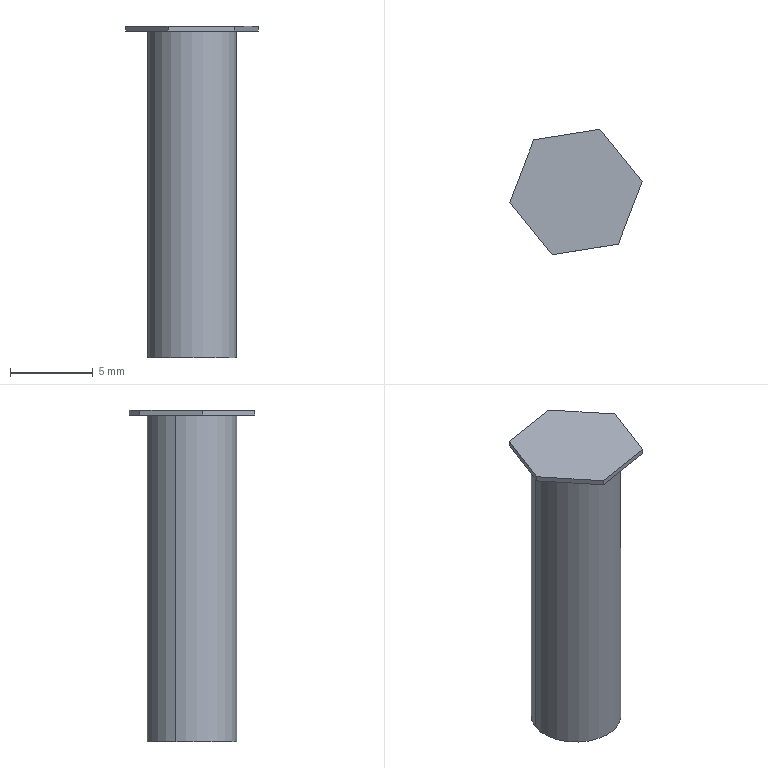Component | SolidWorks | P16BoxWeldment-1_BSO-M3-20-13 | 1 solid | 14 faces | box 7.99 x 7.56 x 20 mm | volume 358 mm3 | plane 10 | cylinder 4 | commonest cylinder face diameters 3 x2 5.4 x2
STEP:
#1=COLOUR_RGB('',0.7922,0.8196,0.9333);
#2=FILL_AREA_STYLE_COLOUR('',#1);
#3=FILL_AREA_STYLE('',(#2));
#4=SURFACE_STYLE_FILL_AREA(#3);
#5=SURFACE_SIDE_STYLE('',(#4));
#6=SURFACE_STYLE_USAGE(.BOTH.,#5);
#7=PRESENTATION_STYLE_ASSIGNMENT((#6));
#8=CARTESIAN_POINT('',(-18.287,3.589,2.535));
#9=VERTEX_POINT('',#8);
#10=CARTESIAN_POINT('',(-18.397,3.632,2.535));
#11=VERTEX_POINT('',#10);
#12=CARTESIAN_POINT('',(-18.342,3.611,2.535));
#13=DIRECTION('',(-0.,0.,-1.));
#14=DIRECTION('',(-0.9339,0.3575,0.));
#15=AXIS2_PLACEMENT_3D('',#12,#13,#14);
#16=CIRCLE('',#15,0.05906);
#17=EDGE_CURVE('',#9,#11,#16,.T.);
#18=ORIENTED_EDGE('',*,*,#17,.F.);
#19=CARTESIAN_POINT('',(-18.287,3.589,1.945));
#20=VERTEX_POINT('',#19);
#21=CARTESIAN_POINT('',(-18.287,3.589,2.535));
#22=DIRECTION('',(-0.,0.,-1.));
#23=VECTOR('',#22,39.37);
#24=LINE('',#21,#23);
#25=EDGE_CURVE('',#9,#20,#24,.T.);
#26=ORIENTED_EDGE('',*,*,#25,.T.);
#27=CARTESIAN_POINT('',(-18.397,3.632,1.945));
#28=VERTEX_POINT('',#27);
#29=CARTESIAN_POINT('',(-18.342,3.611,1.945));
#30=DIRECTION('',(-0.,0.,-1.));
#31=DIRECTION('',(-0.9339,0.3575,0.));
#32=AXIS2_PLACEMENT_3D('',#29,#30,#31);
#33=CIRCLE('',#32,0.05906);
#34=EDGE_CURVE('',#20,#28,#33,.T.);
#35=ORIENTED_EDGE('',*,*,#34,.T.);
#36=CARTESIAN_POINT('',(-18.397,3.632,2.535));
#37=DIRECTION('',(-0.,0.,-1.));
#38=VECTOR('',#37,39.37);
#39=LINE('',#36,#38);
#40=EDGE_CURVE('',#11,#28,#39,.T.);
#41=ORIENTED_EDGE('',*,*,#40,.F.);
#42=EDGE_LOOP('',(#18,#26,#35,#41));
#43=FACE_OUTER_BOUND('',#42,.T.);
#44=CARTESIAN_POINT('',(-18.342,3.611,2.535));
#45=DIRECTION('',(-0.,0.,-1.));
#46=DIRECTION('',(-0.9339,0.3575,0.));
#47=AXIS2_PLACEMENT_3D('',#44,#45,#46);
#48=CYLINDRICAL_SURFACE('',#47,0.05906);
#49=ADVANCED_FACE('',(#43),#48,.F.);
#50=CARTESIAN_POINT('',(-18.442,3.649,1.945));
#51=VERTEX_POINT('',#50);
#52=CARTESIAN_POINT('',(-18.243,3.573,1.945));
#53=VERTEX_POINT('',#52);
#54=CARTESIAN_POINT('',(-18.342,3.611,1.945));
#55=DIRECTION('',(-0.,0.,-1.));
#56=DIRECTION('',(-0.9339,0.3575,0.));
#57=AXIS2_PLACEMENT_3D('',#54,#55,#56);
#58=CIRCLE('',#57,0.1063);
#59=EDGE_CURVE('',#51,#53,#58,.T.);
#60=ORIENTED_EDGE('',*,*,#59,.F.);
#61=CARTESIAN_POINT('',(-18.442,3.649,2.72));
#62=VERTEX_POINT('',#61);
#63=CARTESIAN_POINT('',(-18.442,3.649,1.945));
#64=DIRECTION('',(0.,-0.,1.));
#65=VECTOR('',#64,39.37);
#66=LINE('',#63,#65);
#67=EDGE_CURVE('',#51,#62,#66,.T.);
#68=ORIENTED_EDGE('',*,*,#67,.T.);
#69=CARTESIAN_POINT('',(-18.243,3.573,2.72));
#70=VERTEX_POINT('',#69);
#71=CARTESIAN_POINT('',(-18.342,3.611,2.72));
#72=DIRECTION('',(0.,-0.,1.));
#73=DIRECTION('',(0.9339,-0.3575,0.));
#74=AXIS2_PLACEMENT_3D('',#71,#72,#73);
#75=CIRCLE('',#74,0.1063);
#76=EDGE_CURVE('',#70,#62,#75,.T.);
#77=ORIENTED_EDGE('',*,*,#76,.F.);
#78=CARTESIAN_POINT('',(-18.243,3.573,1.945));
#79=DIRECTION('',(0.,-0.,1.));
#80=VECTOR('',#79,39.37);
#81=LINE('',#78,#80);
#82=EDGE_CURVE('',#53,#70,#81,.T.);
#83=ORIENTED_EDGE('',*,*,#82,.F.);
#84=EDGE_LOOP('',(#60,#68,#77,#83));
#85=FACE_OUTER_BOUND('',#84,.T.);
#86=CARTESIAN_POINT('',(-18.342,3.611,1.945));
#87=DIRECTION('',(0.,-0.,1.));
#88=DIRECTION('',(0.9339,-0.3575,0.));
#89=AXIS2_PLACEMENT_3D('',#86,#87,#88);
#90=CYLINDRICAL_SURFACE('',#89,0.1063);
#91=ADVANCED_FACE('',(#85),#90,.T.);
#92=ORIENTED_EDGE('',*,*,#67,.F.);
#93=CARTESIAN_POINT('',(-18.342,3.611,1.945));
#94=DIRECTION('',(-0.,0.,-1.));
#95=DIRECTION('',(-0.9339,0.3575,0.));
#96=AXIS2_PLACEMENT_3D('',#93,#94,#95);
#97=CIRCLE('',#96,0.1063);
#98=EDGE_CURVE('',#53,#51,#97,.T.);
#99=ORIENTED_EDGE('',*,*,#98,.F.);
#100=ORIENTED_EDGE('',*,*,#82,.T.);
#101=CARTESIAN_POINT('',(-18.342,3.611,2.72));
#102=DIRECTION('',(0.,-0.,1.));
#103=DIRECTION('',(0.9339,-0.3575,0.));
#104=AXIS2_PLACEMENT_3D('',#101,#102,#103);
#105=CIRCLE('',#104,0.1063);
#106=EDGE_CURVE('',#62,#70,#105,.T.);
#107=ORIENTED_EDGE('',*,*,#106,.F.);
#108=EDGE_LOOP('',(#92,#99,#100,#107));
#109=FACE_OUTER_BOUND('',#108,.T.);
#110=CARTESIAN_POINT('',(-18.342,3.611,1.945));
#111=DIRECTION('',(0.,-0.,1.));
#112=DIRECTION('',(0.9339,-0.3575,0.));
#113=AXIS2_PLACEMENT_3D('',#110,#111,#112);
#114=CYLINDRICAL_SURFACE('',#113,0.1063);
#115=ADVANCED_FACE('',(#109),#114,.T.);
#116=CARTESIAN_POINT('',(-18.342,3.611,1.945));
#117=DIRECTION('',(-0.,0.,-1.));
#118=DIRECTION('',(-0.9339,0.3575,0.));
#119=AXIS2_PLACEMENT_3D('',#116,#117,#118);
#120=CIRCLE('',#119,0.05906);
#121=EDGE_CURVE('',#28,#20,#120,.T.);
#122=ORIENTED_EDGE('',*,*,#121,.F.);
#123=ORIENTED_EDGE('',*,*,#34,.F.);
#124=EDGE_LOOP('',(#122,#123));
#125=FACE_BOUND('',#124,.T.);
#126=ORIENTED_EDGE('',*,*,#98,.T.);
#127=ORIENTED_EDGE('',*,*,#59,.T.);
#128=EDGE_LOOP('',(#126,#127));
#129=FACE_OUTER_BOUND('',#128,.T.);
#130=CARTESIAN_POINT('',(-18.342,3.611,1.945));
#131=DIRECTION('',(-0.,0.,-1.));
#132=DIRECTION('',(-0.9339,0.3575,0.));
#133=AXIS2_PLACEMENT_3D('',#130,#131,#132);
#134=PLANE('',#133);
#135=ADVANCED_FACE('',(#125,#129),#134,.T.);
#136=CARTESIAN_POINT('',(-18.5,3.585,2.72));
#137=VERTEX_POINT('',#136);
#138=CARTESIAN_POINT('',(-18.399,3.462,2.72));
#139=VERTEX_POINT('',#138);
#140=CARTESIAN_POINT('',(-18.5,3.585,2.72));
#141=DIRECTION('',(0.63,-0.7766,-0.));
#142=VECTOR('',#141,39.37);
#143=LINE('',#140,#142);
#144=EDGE_CURVE('',#137,#139,#143,.T.);
#145=ORIENTED_EDGE('',*,*,#144,.F.);
#146=CARTESIAN_POINT('',(-18.443,3.734,2.72));
#147=VERTEX_POINT('',#146);
#148=CARTESIAN_POINT('',(-18.443,3.734,2.72));
#149=DIRECTION('',(-0.3575,-0.9339,-0.));
#150=VECTOR('',#149,39.37);
#151=LINE('',#148,#150);
#152=EDGE_CURVE('',#147,#137,#151,.T.);
#153=ORIENTED_EDGE('',*,*,#152,.F.);
#154=CARTESIAN_POINT('',(-18.285,3.759,2.72));
#155=VERTEX_POINT('',#154);
#156=CARTESIAN_POINT('',(-18.285,3.759,2.72));
#157=DIRECTION('',(-0.9875,-0.1573,0.));
#158=VECTOR('',#157,39.37);
#159=LINE('',#156,#158);
#160=EDGE_CURVE('',#155,#147,#159,.T.);
#161=ORIENTED_EDGE('',*,*,#160,.F.);
#162=CARTESIAN_POINT('',(-18.185,3.636,2.72));
#163=VERTEX_POINT('',#162);
#164=CARTESIAN_POINT('',(-18.185,3.636,2.72));
#165=DIRECTION('',(-0.63,0.7766,0.));
#166=VECTOR('',#165,39.37);
#167=LINE('',#164,#166);
#168=EDGE_CURVE('',#163,#155,#167,.T.);
#169=ORIENTED_EDGE('',*,*,#168,.F.);
#170=CARTESIAN_POINT('',(-18.242,3.487,2.72));
#171=VERTEX_POINT('',#170);
#172=CARTESIAN_POINT('',(-18.242,3.487,2.72));
#173=DIRECTION('',(0.3575,0.9339,0.));
#174=VECTOR('',#173,39.37);
#175=LINE('',#172,#174);
#176=EDGE_CURVE('',#171,#163,#175,.T.);
#177=ORIENTED_EDGE('',*,*,#176,.F.);
#178=CARTESIAN_POINT('',(-18.399,3.462,2.72));
#179=DIRECTION('',(0.9875,0.1573,-0.));
#180=VECTOR('',#179,39.37);
#181=LINE('',#178,#180);
#182=EDGE_CURVE('',#139,#171,#181,.T.);
#183=ORIENTED_EDGE('',*,*,#182,.F.);
#184=EDGE_LOOP('',(#145,#153,#161,#169,#177,#183));
#185=FACE_OUTER_BOUND('',#184,.T.);
#186=ORIENTED_EDGE('',*,*,#76,.T.);
#187=ORIENTED_EDGE('',*,*,#106,.T.);
#188=EDGE_LOOP('',(#186,#187));
#189=FACE_BOUND('',#188,.T.);
#190=CARTESIAN_POINT('',(-18.342,3.611,2.72));
#191=DIRECTION('',(0.,-0.,1.));
#192=DIRECTION('',(0.9339,-0.3575,-0.));
#193=AXIS2_PLACEMENT_3D('',#190,#191,#192);
#194=PLANE('',#193);
#195=ADVANCED_FACE('',(#185,#189),#194,.F.);
#196=CARTESIAN_POINT('',(-18.5,3.585,2.732));
#197=VERTEX_POINT('',#196);
#198=CARTESIAN_POINT('',(-18.399,3.462,2.732));
#199=VERTEX_POINT('',#198);
#200=CARTESIAN_POINT('',(-18.5,3.585,2.732));
#201=DIRECTION('',(0.63,-0.7766,-0.));
#202=VECTOR('',#201,39.37);
#203=LINE('',#200,#202);
#204=EDGE_CURVE('',#197,#199,#203,.T.);
#205=ORIENTED_EDGE('',*,*,#204,.F.);
#206=CARTESIAN_POINT('',(-18.5,3.585,2.72));
#207=DIRECTION('',(0.,-0.,1.));
#208=VECTOR('',#207,39.37);
#209=LINE('',#206,#208);
#210=EDGE_CURVE('',#137,#197,#209,.T.);
#211=ORIENTED_EDGE('',*,*,#210,.F.);
#212=ORIENTED_EDGE('',*,*,#144,.T.);
#213=CARTESIAN_POINT('',(-18.399,3.462,2.72));
#214=DIRECTION('',(0.,-0.,1.));
#215=VECTOR('',#214,39.37);
#216=LINE('',#213,#215);
#217=EDGE_CURVE('',#139,#199,#216,.T.);
#218=ORIENTED_EDGE('',*,*,#217,.T.);
#219=EDGE_LOOP('',(#205,#211,#212,#218));
#220=FACE_OUTER_BOUND('',#219,.T.);
#221=CARTESIAN_POINT('',(-18.5,3.585,2.72));
#222=DIRECTION('',(-0.7766,-0.63,0.));
#223=DIRECTION('',(-0.63,0.7766,0.));
#224=AXIS2_PLACEMENT_3D('',#221,#222,#223);
#225=PLANE('',#224);
#226=ADVANCED_FACE('',(#220),#225,.T.);
#227=CARTESIAN_POINT('',(-18.443,3.734,2.732));
#228=VERTEX_POINT('',#227);
#229=CARTESIAN_POINT('',(-18.443,3.734,2.732));
#230=DIRECTION('',(-0.3575,-0.9339,-0.));
#231=VECTOR('',#230,39.37);
#232=LINE('',#229,#231);
#233=EDGE_CURVE('',#228,#197,#232,.T.);
#234=ORIENTED_EDGE('',*,*,#233,.F.);
#235=CARTESIAN_POINT('',(-18.443,3.734,2.72));
#236=DIRECTION('',(0.,-0.,1.));
#237=VECTOR('',#236,39.37);
#238=LINE('',#235,#237);
#239=EDGE_CURVE('',#147,#228,#238,.T.);
#240=ORIENTED_EDGE('',*,*,#239,.F.);
#241=ORIENTED_EDGE('',*,*,#152,.T.);
#242=ORIENTED_EDGE('',*,*,#210,.T.);
#243=EDGE_LOOP('',(#234,#240,#241,#242));
#244=FACE_OUTER_BOUND('',#243,.T.);
#245=CARTESIAN_POINT('',(-18.443,3.734,2.72));
#246=DIRECTION('',(-0.9339,0.3575,0.));
#247=DIRECTION('',(0.3575,0.9339,0.));
#248=AXIS2_PLACEMENT_3D('',#245,#246,#247);
#249=PLANE('',#248);
#250=ADVANCED_FACE('',(#244),#249,.T.);
#251=CARTESIAN_POINT('',(-18.285,3.759,2.732));
#252=VERTEX_POINT('',#251);
#253=CARTESIAN_POINT('',(-18.285,3.759,2.732));
#254=DIRECTION('',(-0.9875,-0.1573,0.));
#255=VECTOR('',#254,39.37);
#256=LINE('',#253,#255);
#257=EDGE_CURVE('',#252,#228,#256,.T.);
#258=ORIENTED_EDGE('',*,*,#257,.F.);
#259=CARTESIAN_POINT('',(-18.285,3.759,2.72));
#260=DIRECTION('',(0.,-0.,1.));
#261=VECTOR('',#260,39.37);
#262=LINE('',#259,#261);
#263=EDGE_CURVE('',#155,#252,#262,.T.);
#264=ORIENTED_EDGE('',*,*,#263,.F.);
#265=ORIENTED_EDGE('',*,*,#160,.T.);
#266=ORIENTED_EDGE('',*,*,#239,.T.);
#267=EDGE_LOOP('',(#258,#264,#265,#266));
#268=FACE_OUTER_BOUND('',#267,.T.);
#269=CARTESIAN_POINT('',(-18.285,3.759,2.72));
#270=DIRECTION('',(-0.1573,0.9875,0.));
#271=DIRECTION('',(0.9875,0.1573,-0.));
#272=AXIS2_PLACEMENT_3D('',#269,#270,#271);
#273=PLANE('',#272);
#274=ADVANCED_FACE('',(#268),#273,.T.);
#275=CARTESIAN_POINT('',(-18.185,3.636,2.732));
#276=VERTEX_POINT('',#275);
#277=CARTESIAN_POINT('',(-18.185,3.636,2.732));
#278=DIRECTION('',(-0.63,0.7766,0.));
#279=VECTOR('',#278,39.37);
#280=LINE('',#277,#279);
#281=EDGE_CURVE('',#276,#252,#280,.T.);
#282=ORIENTED_EDGE('',*,*,#281,.F.);
#283=CARTESIAN_POINT('',(-18.185,3.636,2.72));
#284=DIRECTION('',(0.,-0.,1.));
#285=VECTOR('',#284,39.37);
#286=LINE('',#283,#285);
#287=EDGE_CURVE('',#163,#276,#286,.T.);
#288=ORIENTED_EDGE('',*,*,#287,.F.);
#289=ORIENTED_EDGE('',*,*,#168,.T.);
#290=ORIENTED_EDGE('',*,*,#263,.T.);
#291=EDGE_LOOP('',(#282,#288,#289,#290));
#292=FACE_OUTER_BOUND('',#291,.T.);
#293=CARTESIAN_POINT('',(-18.185,3.636,2.72));
#294=DIRECTION('',(0.7766,0.63,-0.));
#295=DIRECTION('',(0.63,-0.7766,-0.));
#296=AXIS2_PLACEMENT_3D('',#293,#294,#295);
#297=PLANE('',#296);
#298=ADVANCED_FACE('',(#292),#297,.T.);
#299=CARTESIAN_POINT('',(-18.242,3.487,2.732));
#300=VERTEX_POINT('',#299);
#301=CARTESIAN_POINT('',(-18.242,3.487,2.732));
#302=DIRECTION('',(0.3575,0.9339,0.));
#303=VECTOR('',#302,39.37);
#304=LINE('',#301,#303);
#305=EDGE_CURVE('',#300,#276,#304,.T.);
#306=ORIENTED_EDGE('',*,*,#305,.F.);
#307=CARTESIAN_POINT('',(-18.242,3.487,2.72));
#308=DIRECTION('',(0.,-0.,1.));
#309=VECTOR('',#308,39.37);
#310=LINE('',#307,#309);
#311=EDGE_CURVE('',#171,#300,#310,.T.);
#312=ORIENTED_EDGE('',*,*,#311,.F.);
#313=ORIENTED_EDGE('',*,*,#176,.T.);
#314=ORIENTED_EDGE('',*,*,#287,.T.);
#315=EDGE_LOOP('',(#306,#312,#313,#314));
#316=FACE_OUTER_BOUND('',#315,.T.);
#317=CARTESIAN_POINT('',(-18.242,3.487,2.72));
#318=DIRECTION('',(0.9339,-0.3575,-0.));
#319=DIRECTION('',(-0.3575,-0.9339,-0.));
#320=AXIS2_PLACEMENT_3D('',#317,#318,#319);
#321=PLANE('',#320);
#322=ADVANCED_FACE('',(#316),#321,.T.);
#323=CARTESIAN_POINT('',(-18.399,3.462,2.732));
#324=DIRECTION('',(0.9875,0.1573,-0.));
#325=VECTOR('',#324,39.37);
#326=LINE('',#323,#325);
#327=EDGE_CURVE('',#199,#300,#326,.T.);
#328=ORIENTED_EDGE('',*,*,#327,.F.);
#329=ORIENTED_EDGE('',*,*,#217,.F.);
#330=ORIENTED_EDGE('',*,*,#182,.T.);
#331=ORIENTED_EDGE('',*,*,#311,.T.);
#332=EDGE_LOOP('',(#328,#329,#330,#331));
#333=FACE_OUTER_BOUND('',#332,.T.);
#334=CARTESIAN_POINT('',(-18.399,3.462,2.72));
#335=DIRECTION('',(0.1573,-0.9875,-0.));
#336=DIRECTION('',(-0.9875,-0.1573,0.));
#337=AXIS2_PLACEMENT_3D('',#334,#335,#336);
#338=PLANE('',#337);
#339=ADVANCED_FACE('',(#333),#338,.T.);
#340=ORIENTED_EDGE('',*,*,#204,.T.);
#341=ORIENTED_EDGE('',*,*,#327,.T.);
#342=ORIENTED_EDGE('',*,*,#305,.T.);
#343=ORIENTED_EDGE('',*,*,#281,.T.);
#344=ORIENTED_EDGE('',*,*,#257,.T.);
#345=ORIENTED_EDGE('',*,*,#233,.T.);
#346=EDGE_LOOP('',(#340,#341,#342,#343,#344,#345));
#347=FACE_OUTER_BOUND('',#346,.T.);
#348=CARTESIAN_POINT('',(-18.342,3.611,2.732));
#349=DIRECTION('',(-0.,0.,-1.));
#350=DIRECTION('',(-0.9339,0.3575,0.));
#351=AXIS2_PLACEMENT_3D('',#348,#349,#350);
#352=PLANE('',#351);
#353=ADVANCED_FACE('',(#347),#352,.F.);
#354=ORIENTED_EDGE('',*,*,#25,.F.);
#355=CARTESIAN_POINT('',(-18.342,3.611,2.535));
#356=DIRECTION('',(-0.,0.,-1.));
#357=DIRECTION('',(-0.9339,0.3575,0.));
#358=AXIS2_PLACEMENT_3D('',#355,#356,#357);
#359=CIRCLE('',#358,0.05906);
#360=EDGE_CURVE('',#11,#9,#359,.T.);
#361=ORIENTED_EDGE('',*,*,#360,.F.);
#362=ORIENTED_EDGE('',*,*,#40,.T.);
#363=ORIENTED_EDGE('',*,*,#121,.T.);
#364=EDGE_LOOP('',(#354,#361,#362,#363));
#365=FACE_OUTER_BOUND('',#364,.T.);
#366=CARTESIAN_POINT('',(-18.342,3.611,2.535));
#367=DIRECTION('',(-0.,0.,-1.));
#368=DIRECTION('',(-0.9339,0.3575,0.));
#369=AXIS2_PLACEMENT_3D('',#366,#367,#368);
#370=CYLINDRICAL_SURFACE('',#369,0.05906);
#371=ADVANCED_FACE('',(#365),#370,.F.);
#372=ORIENTED_EDGE('',*,*,#360,.T.);
#373=ORIENTED_EDGE('',*,*,#17,.T.);
#374=EDGE_LOOP('',(#372,#373));
#375=FACE_OUTER_BOUND('',#374,.T.);
#376=CARTESIAN_POINT('',(-18.342,3.611,2.535));
#377=DIRECTION('',(-0.,0.,-1.));
#378=DIRECTION('',(-0.9339,0.3575,0.));
#379=AXIS2_PLACEMENT_3D('',#376,#377,#378);
#380=PLANE('',#379);
#381=ADVANCED_FACE('',(#375),#380,.T.);
#382=CLOSED_SHELL('',(#49,#91,#115,#135,#195,#226,#250,#274,#298,#322,#339,#353,#371,#381));
#383=MANIFOLD_SOLID_BREP('',#382);
#384=STYLED_ITEM('',(#7),#383);
#385=(LENGTH_UNIT()NAMED_UNIT(*)SI_UNIT($,.METRE.));
#386=LENGTH_MEASURE_WITH_UNIT(LENGTH_MEASURE(0.0254),#385);
#387=DIMENSIONAL_EXPONENTS(1.,0.,0.,0.,0.,0.,0.);
#388=(CONVERSION_BASED_UNIT('',#386)LENGTH_UNIT()NAMED_UNIT(#387));
#389=UNCERTAINTY_MEASURE_WITH_UNIT(LENGTH_MEASURE(0.00001),#388,'','');
#390=(NAMED_UNIT(*)PLANE_ANGLE_UNIT()SI_UNIT($,.RADIAN.));
#391=(NAMED_UNIT(*)SI_UNIT($,.STERADIAN.)SOLID_ANGLE_UNIT());
#392=(GEOMETRIC_REPRESENTATION_CONTEXT(3)GLOBAL_UNCERTAINTY_ASSIGNED_CONTEXT((#389))GLOBAL_UNIT_ASSIGNED_CONTEXT((#388,#390,#391))REPRESENTATION_CONTEXT('',''));
#393=MECHANICAL_DESIGN_GEOMETRIC_PRESENTATION_REPRESENTATION('',(#384),#392);
#394=CARTESIAN_POINT('',(0.,0.,0.));
#395=DIRECTION('',(0.,0.,1.));
#396=DIRECTION('',(1.,0.,0.));
#397=AXIS2_PLACEMENT_3D('',#394,#395,#396);
#398=(LENGTH_UNIT()NAMED_UNIT(*)SI_UNIT($,.METRE.));
#399=LENGTH_MEASURE_WITH_UNIT(LENGTH_MEASURE(0.0254),#398);
#400=DIMENSIONAL_EXPONENTS(1.,0.,0.,0.,0.,0.,0.);
#401=(CONVERSION_BASED_UNIT('',#399)LENGTH_UNIT()NAMED_UNIT(#400));
#402=UNCERTAINTY_MEASURE_WITH_UNIT(LENGTH_MEASURE(0.00001),#401,'','');
#403=(NAMED_UNIT(*)PLANE_ANGLE_UNIT()SI_UNIT($,.RADIAN.));
#404=(NAMED_UNIT(*)SI_UNIT($,.STERADIAN.)SOLID_ANGLE_UNIT());
#405=(GEOMETRIC_REPRESENTATION_CONTEXT(3)GLOBAL_UNCERTAINTY_ASSIGNED_CONTEXT((#402))GLOBAL_UNIT_ASSIGNED_CONTEXT((#401,#403,#404))REPRESENTATION_CONTEXT('',''));
#406=ADVANCED_BREP_SHAPE_REPRESENTATION('',(#383,#397),#405);
#407=PRESENTATION_LAYER_ASSIGNMENT('','',(#384));